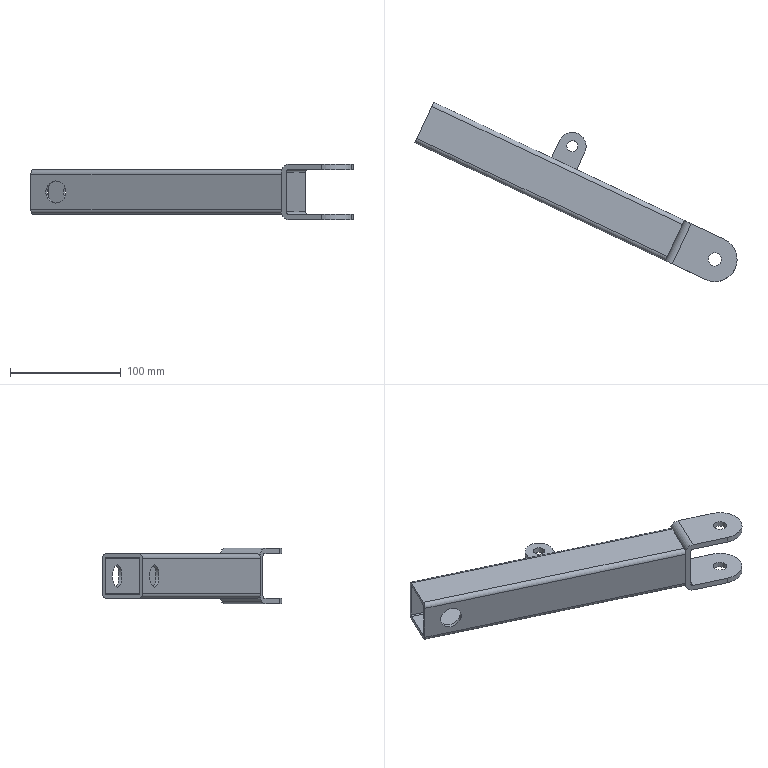Component | SolidWorks | FilmPressingSoilCoveringMechanism2Reverse-2_PressingFilmSoilPlateMovableFrame-1 | 2 solids | 58 faces | volume 140320 mm3 | cylinder 32 | plane 26 | commonest cylinder face diameters 10 x4 20 x4 8 x4 2 x4 25 x4 12 x4 40 x4 4 x2